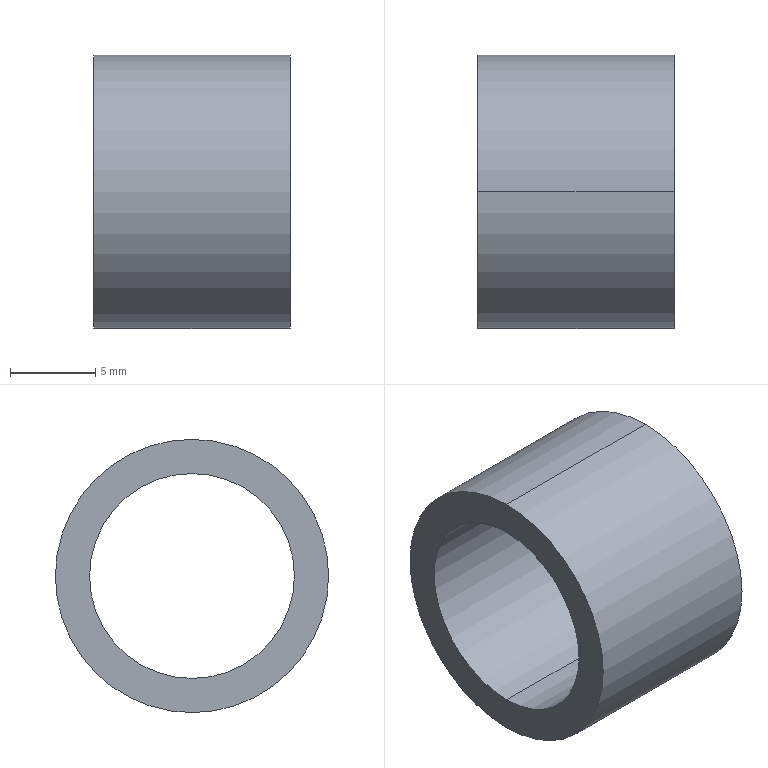Component | SolidWorks | GearBushing-2 | 1 solid | 6 faces | box 11.5 x 16 x 16 mm | volume 1012 mm3 | cylinder 4 | plane 2 | commonest cylinder face diameters 12 x2 16 x2
build123d program:
from build123d import *

# Parameters (mm, degrees)
SKETCH1_R           = 8
SKETCH1_R_2         = 6
BOSS_EXTRUDE1_DEPTH = 11.5


with BuildPart() as part:
    # Sketch1 → Boss-Extrude1 (new body)
    with BuildSketch(Plane.XY):
        with Locations((64.2, 0)):
            Circle(SKETCH1_R)
        with Locations((64.2, 0)):
            Circle(SKETCH1_R_2, mode=Mode.SUBTRACT)
    extrude(amount=BOSS_EXTRUDE1_DEPTH)


solid = part.part

# Placed as in the assembly
solid = solid.moved(Location((-5.375, -67.172, 107.182), (0, 90, 0)))
STEP:
#1=COLOUR_RGB('',0.7922,0.8196,0.9333);
#2=FILL_AREA_STYLE_COLOUR('',#1);
#3=FILL_AREA_STYLE('',(#2));
#4=SURFACE_STYLE_FILL_AREA(#3);
#5=SURFACE_SIDE_STYLE('',(#4));
#6=SURFACE_STYLE_USAGE(.BOTH.,#5);
#7=PRESENTATION_STYLE_ASSIGNMENT((#6));
#8=CARTESIAN_POINT('',(0.2411,-2.645,1.456));
#9=VERTEX_POINT('',#8);
#10=CARTESIAN_POINT('',(0.2411,-2.644,1.928));
#11=VERTEX_POINT('',#10);
#12=CARTESIAN_POINT('',(0.2411,-2.645,1.692));
#13=DIRECTION('',(1.,-0.,-0.));
#14=DIRECTION('',(0.,0.001768,1.));
#15=AXIS2_PLACEMENT_3D('',#12,#13,#14);
#16=CIRCLE('',#15,0.2362);
#17=EDGE_CURVE('',#9,#11,#16,.T.);
#18=ORIENTED_EDGE('',*,*,#17,.T.);
#19=CARTESIAN_POINT('',(-0.2116,-2.644,1.928));
#20=VERTEX_POINT('',#19);
#21=CARTESIAN_POINT('',(0.2411,-2.644,1.928));
#22=DIRECTION('',(-1.,0.,0.));
#23=VECTOR('',#22,39.37);
#24=LINE('',#21,#23);
#25=EDGE_CURVE('',#11,#20,#24,.T.);
#26=ORIENTED_EDGE('',*,*,#25,.T.);
#27=CARTESIAN_POINT('',(-0.2116,-2.645,1.456));
#28=VERTEX_POINT('',#27);
#29=CARTESIAN_POINT('',(-0.2116,-2.645,1.692));
#30=DIRECTION('',(1.,-0.,-0.));
#31=DIRECTION('',(0.,0.001768,1.));
#32=AXIS2_PLACEMENT_3D('',#29,#30,#31);
#33=CIRCLE('',#32,0.2362);
#34=EDGE_CURVE('',#28,#20,#33,.T.);
#35=ORIENTED_EDGE('',*,*,#34,.F.);
#36=CARTESIAN_POINT('',(0.2411,-2.645,1.456));
#37=DIRECTION('',(-1.,0.,0.));
#38=VECTOR('',#37,39.37);
#39=LINE('',#36,#38);
#40=EDGE_CURVE('',#9,#28,#39,.T.);
#41=ORIENTED_EDGE('',*,*,#40,.F.);
#42=EDGE_LOOP('',(#18,#26,#35,#41));
#43=FACE_OUTER_BOUND('',#42,.T.);
#44=CARTESIAN_POINT('',(0.2411,-2.645,1.692));
#45=DIRECTION('',(-1.,0.,0.));
#46=DIRECTION('',(0.,-0.001768,-1.));
#47=AXIS2_PLACEMENT_3D('',#44,#45,#46);
#48=CYLINDRICAL_SURFACE('',#47,0.2362);
#49=ADVANCED_FACE('',(#43),#48,.F.);
#50=CARTESIAN_POINT('',(0.2411,-2.644,2.007));
#51=VERTEX_POINT('',#50);
#52=CARTESIAN_POINT('',(0.2411,-2.645,1.377));
#53=VERTEX_POINT('',#52);
#54=CARTESIAN_POINT('',(0.2411,-2.645,1.692));
#55=DIRECTION('',(1.,-0.,-0.));
#56=DIRECTION('',(0.,0.001768,1.));
#57=AXIS2_PLACEMENT_3D('',#54,#55,#56);
#58=CIRCLE('',#57,0.315);
#59=EDGE_CURVE('',#51,#53,#58,.T.);
#60=ORIENTED_EDGE('',*,*,#59,.F.);
#61=CARTESIAN_POINT('',(-0.2116,-2.644,2.007));
#62=VERTEX_POINT('',#61);
#63=CARTESIAN_POINT('',(0.2411,-2.644,2.007));
#64=DIRECTION('',(-1.,0.,0.));
#65=VECTOR('',#64,39.37);
#66=LINE('',#63,#65);
#67=EDGE_CURVE('',#51,#62,#66,.T.);
#68=ORIENTED_EDGE('',*,*,#67,.T.);
#69=CARTESIAN_POINT('',(-0.2116,-2.645,1.377));
#70=VERTEX_POINT('',#69);
#71=CARTESIAN_POINT('',(-0.2116,-2.645,1.692));
#72=DIRECTION('',(1.,-0.,-0.));
#73=DIRECTION('',(0.,0.001768,1.));
#74=AXIS2_PLACEMENT_3D('',#71,#72,#73);
#75=CIRCLE('',#74,0.315);
#76=EDGE_CURVE('',#62,#70,#75,.T.);
#77=ORIENTED_EDGE('',*,*,#76,.T.);
#78=CARTESIAN_POINT('',(0.2411,-2.645,1.377));
#79=DIRECTION('',(-1.,0.,0.));
#80=VECTOR('',#79,39.37);
#81=LINE('',#78,#80);
#82=EDGE_CURVE('',#53,#70,#81,.T.);
#83=ORIENTED_EDGE('',*,*,#82,.F.);
#84=EDGE_LOOP('',(#60,#68,#77,#83));
#85=FACE_OUTER_BOUND('',#84,.T.);
#86=CARTESIAN_POINT('',(0.2411,-2.645,1.692));
#87=DIRECTION('',(-1.,0.,0.));
#88=DIRECTION('',(0.,-0.001768,-1.));
#89=AXIS2_PLACEMENT_3D('',#86,#87,#88);
#90=CYLINDRICAL_SURFACE('',#89,0.315);
#91=ADVANCED_FACE('',(#85),#90,.T.);
#92=CARTESIAN_POINT('',(0.2411,-2.645,1.692));
#93=DIRECTION('',(1.,-0.,-0.));
#94=DIRECTION('',(0.,0.001768,1.));
#95=AXIS2_PLACEMENT_3D('',#92,#93,#94);
#96=CIRCLE('',#95,0.315);
#97=EDGE_CURVE('',#53,#51,#96,.T.);
#98=ORIENTED_EDGE('',*,*,#97,.T.);
#99=ORIENTED_EDGE('',*,*,#59,.T.);
#100=EDGE_LOOP('',(#98,#99));
#101=FACE_OUTER_BOUND('',#100,.T.);
#102=ORIENTED_EDGE('',*,*,#17,.F.);
#103=CARTESIAN_POINT('',(0.2411,-2.645,1.692));
#104=DIRECTION('',(1.,-0.,-0.));
#105=DIRECTION('',(0.,0.001768,1.));
#106=AXIS2_PLACEMENT_3D('',#103,#104,#105);
#107=CIRCLE('',#106,0.2362);
#108=EDGE_CURVE('',#11,#9,#107,.T.);
#109=ORIENTED_EDGE('',*,*,#108,.F.);
#110=EDGE_LOOP('',(#102,#109));
#111=FACE_BOUND('',#110,.T.);
#112=CARTESIAN_POINT('',(0.2411,-2.645,1.692));
#113=DIRECTION('',(1.,-0.,-0.));
#114=DIRECTION('',(0.,0.001768,1.));
#115=AXIS2_PLACEMENT_3D('',#112,#113,#114);
#116=PLANE('',#115);
#117=ADVANCED_FACE('',(#101,#111),#116,.T.);
#118=CARTESIAN_POINT('',(-0.2116,-2.645,1.692));
#119=DIRECTION('',(1.,-0.,-0.));
#120=DIRECTION('',(0.,0.001768,1.));
#121=AXIS2_PLACEMENT_3D('',#118,#119,#120);
#122=CIRCLE('',#121,0.315);
#123=EDGE_CURVE('',#70,#62,#122,.T.);
#124=ORIENTED_EDGE('',*,*,#123,.F.);
#125=ORIENTED_EDGE('',*,*,#76,.F.);
#126=EDGE_LOOP('',(#124,#125));
#127=FACE_OUTER_BOUND('',#126,.T.);
#128=ORIENTED_EDGE('',*,*,#34,.T.);
#129=CARTESIAN_POINT('',(-0.2116,-2.645,1.692));
#130=DIRECTION('',(1.,-0.,-0.));
#131=DIRECTION('',(0.,0.001768,1.));
#132=AXIS2_PLACEMENT_3D('',#129,#130,#131);
#133=CIRCLE('',#132,0.2362);
#134=EDGE_CURVE('',#20,#28,#133,.T.);
#135=ORIENTED_EDGE('',*,*,#134,.T.);
#136=EDGE_LOOP('',(#128,#135));
#137=FACE_BOUND('',#136,.T.);
#138=CARTESIAN_POINT('',(-0.2116,-2.645,1.692));
#139=DIRECTION('',(1.,-0.,-0.));
#140=DIRECTION('',(0.,0.001768,1.));
#141=AXIS2_PLACEMENT_3D('',#138,#139,#140);
#142=PLANE('',#141);
#143=ADVANCED_FACE('',(#127,#137),#142,.F.);
#144=ORIENTED_EDGE('',*,*,#67,.F.);
#145=ORIENTED_EDGE('',*,*,#97,.F.);
#146=ORIENTED_EDGE('',*,*,#82,.T.);
#147=ORIENTED_EDGE('',*,*,#123,.T.);
#148=EDGE_LOOP('',(#144,#145,#146,#147));
#149=FACE_OUTER_BOUND('',#148,.T.);
#150=CARTESIAN_POINT('',(0.2411,-2.645,1.692));
#151=DIRECTION('',(-1.,0.,0.));
#152=DIRECTION('',(0.,-0.001768,-1.));
#153=AXIS2_PLACEMENT_3D('',#150,#151,#152);
#154=CYLINDRICAL_SURFACE('',#153,0.315);
#155=ADVANCED_FACE('',(#149),#154,.T.);
#156=ORIENTED_EDGE('',*,*,#25,.F.);
#157=ORIENTED_EDGE('',*,*,#108,.T.);
#158=ORIENTED_EDGE('',*,*,#40,.T.);
#159=ORIENTED_EDGE('',*,*,#134,.F.);
#160=EDGE_LOOP('',(#156,#157,#158,#159));
#161=FACE_OUTER_BOUND('',#160,.T.);
#162=CARTESIAN_POINT('',(0.2411,-2.645,1.692));
#163=DIRECTION('',(-1.,0.,0.));
#164=DIRECTION('',(0.,-0.001768,-1.));
#165=AXIS2_PLACEMENT_3D('',#162,#163,#164);
#166=CYLINDRICAL_SURFACE('',#165,0.2362);
#167=ADVANCED_FACE('',(#161),#166,.F.);
#168=CLOSED_SHELL('',(#49,#91,#117,#143,#155,#167));
#169=MANIFOLD_SOLID_BREP('',#168);
#170=STYLED_ITEM('',(#7),#169);
#171=PRESENTATION_LAYER_ASSIGNMENT('','',(#170));
#172=CARTESIAN_POINT('',(0.,0.,0.));
#173=DIRECTION('',(0.,0.,1.));
#174=DIRECTION('',(1.,0.,0.));
#175=AXIS2_PLACEMENT_3D('',#172,#173,#174);
#176=(LENGTH_UNIT()NAMED_UNIT(*)SI_UNIT($,.METRE.));
#177=LENGTH_MEASURE_WITH_UNIT(LENGTH_MEASURE(0.0254),#176);
#178=DIMENSIONAL_EXPONENTS(1.,0.,0.,0.,0.,0.,0.);
#179=(CONVERSION_BASED_UNIT('',#177)LENGTH_UNIT()NAMED_UNIT(#178));
#180=UNCERTAINTY_MEASURE_WITH_UNIT(LENGTH_MEASURE(0.00001),#179,'','');
#181=(NAMED_UNIT(*)PLANE_ANGLE_UNIT()SI_UNIT($,.RADIAN.));
#182=(NAMED_UNIT(*)SI_UNIT($,.STERADIAN.)SOLID_ANGLE_UNIT());
#183=(GEOMETRIC_REPRESENTATION_CONTEXT(3)GLOBAL_UNCERTAINTY_ASSIGNED_CONTEXT((#180))GLOBAL_UNIT_ASSIGNED_CONTEXT((#179,#181,#182))REPRESENTATION_CONTEXT('',''));
#184=ADVANCED_BREP_SHAPE_REPRESENTATION('',(#169,#175),#183);
#185=(LENGTH_UNIT()NAMED_UNIT(*)SI_UNIT($,.METRE.));
#186=LENGTH_MEASURE_WITH_UNIT(LENGTH_MEASURE(0.0254),#185);
#187=DIMENSIONAL_EXPONENTS(1.,0.,0.,0.,0.,0.,0.);
#188=(CONVERSION_BASED_UNIT('',#186)LENGTH_UNIT()NAMED_UNIT(#187));
#189=UNCERTAINTY_MEASURE_WITH_UNIT(LENGTH_MEASURE(0.00001),#188,'','');
#190=(NAMED_UNIT(*)PLANE_ANGLE_UNIT()SI_UNIT($,.RADIAN.));
#191=(NAMED_UNIT(*)SI_UNIT($,.STERADIAN.)SOLID_ANGLE_UNIT());
#192=(GEOMETRIC_REPRESENTATION_CONTEXT(3)GLOBAL_UNCERTAINTY_ASSIGNED_CONTEXT((#189))GLOBAL_UNIT_ASSIGNED_CONTEXT((#188,#190,#191))REPRESENTATION_CONTEXT('',''));
#193=MECHANICAL_DESIGN_GEOMETRIC_PRESENTATION_REPRESENTATION('',(#170),#192);